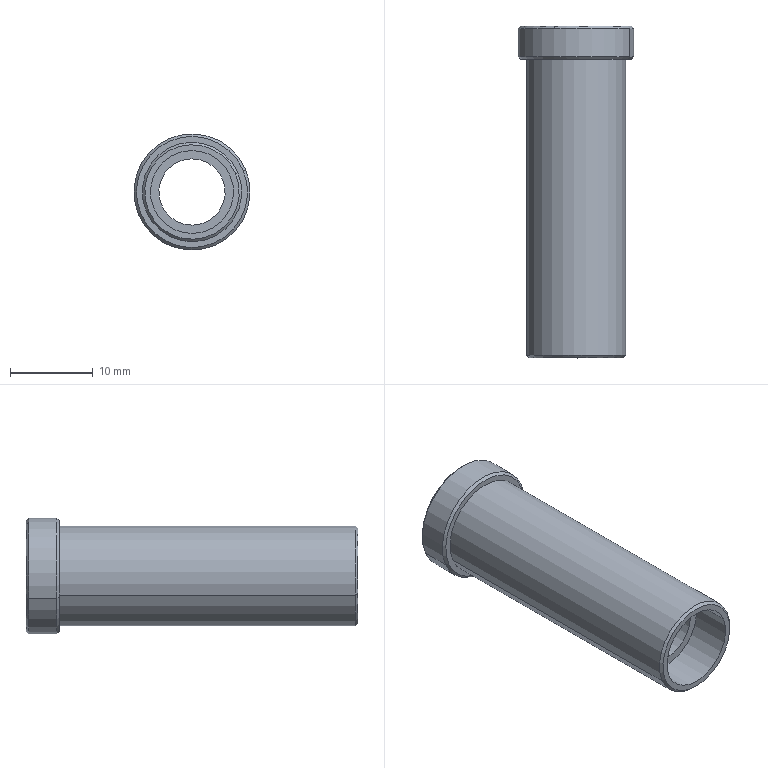Component | SolidWorks | 04LowerMaterialReceivingSwingAngleAssembly(3920)-1_EwellixBallBushingLOC71-D8-L40-E40-G30-7_LOC71-D8-L40-E40-G30-2-1 | 1 solid | 21 faces | box 14 x 40 x 14 mm | volume 2388 mm3 | cylinder 10 | cone 6 | plane 5 | commonest cylinder face diameters 10 x4 12 x2 14 x2 8 x2
STEP:
#1=CARTESIAN_POINT('',(-4.662,5.201,11.122));
#2=VERTEX_POINT('',#1);
#3=CARTESIAN_POINT('',(-5.099,5.201,10.941));
#4=VERTEX_POINT('',#3);
#5=CARTESIAN_POINT('',(-4.88,5.201,11.031));
#6=DIRECTION('',(0.,1.,0.));
#7=DIRECTION('',(0.9237,0.,0.3832));
#8=AXIS2_PLACEMENT_3D('',#5,#6,#7);
#9=CIRCLE('',#8,0.2362);
#10=EDGE_CURVE('',#2,#4,#9,.T.);
#11=ORIENTED_EDGE('',*,*,#10,.T.);
#12=CARTESIAN_POINT('',(-5.099,6.607,10.941));
#13=VERTEX_POINT('',#12);
#14=CARTESIAN_POINT('',(-5.099,-12.921,10.941));
#15=DIRECTION('',(0.,1.,0.));
#16=VECTOR('',#15,39.37);
#17=LINE('',#14,#16);
#18=EDGE_CURVE('',#4,#13,#17,.T.);
#19=ORIENTED_EDGE('',*,*,#18,.T.);
#20=CARTESIAN_POINT('',(-4.662,6.607,11.122));
#21=VERTEX_POINT('',#20);
#22=CARTESIAN_POINT('',(-4.88,6.607,11.031));
#23=DIRECTION('',(-0.,-1.,-0.));
#24=DIRECTION('',(0.9237,0.,0.3832));
#25=AXIS2_PLACEMENT_3D('',#22,#23,#24);
#26=CIRCLE('',#25,0.2362);
#27=EDGE_CURVE('',#13,#21,#26,.T.);
#28=ORIENTED_EDGE('',*,*,#27,.T.);
#29=CARTESIAN_POINT('',(-4.662,-12.921,11.122));
#30=DIRECTION('',(0.,1.,0.));
#31=VECTOR('',#30,39.37);
#32=LINE('',#29,#31);
#33=EDGE_CURVE('',#2,#21,#32,.T.);
#34=ORIENTED_EDGE('',*,*,#33,.F.);
#35=EDGE_LOOP('',(#11,#19,#28,#34));
#36=FACE_OUTER_BOUND('',#35,.T.);
#37=CARTESIAN_POINT('',(-4.88,-12.921,11.031));
#38=DIRECTION('',(0.,1.,0.));
#39=DIRECTION('',(0.9237,0.,0.3832));
#40=AXIS2_PLACEMENT_3D('',#37,#38,#39);
#41=CYLINDRICAL_SURFACE('',#40,0.2362);
#42=ADVANCED_FACE('',(#36),#41,.T.);
#43=CARTESIAN_POINT('',(-4.673,5.189,11.117));
#44=VERTEX_POINT('',#43);
#45=CARTESIAN_POINT('',(-5.088,5.189,10.945));
#46=VERTEX_POINT('',#45);
#47=CARTESIAN_POINT('',(-4.88,5.189,11.031));
#48=DIRECTION('',(0.,1.,0.));
#49=DIRECTION('',(0.9237,0.,0.3832));
#50=AXIS2_PLACEMENT_3D('',#47,#48,#49);
#51=CIRCLE('',#50,0.2244);
#52=EDGE_CURVE('',#44,#46,#51,.T.);
#53=ORIENTED_EDGE('',*,*,#52,.T.);
#54=CARTESIAN_POINT('',(-5.099,5.201,10.941));
#55=DIRECTION('',(-0.6531,0.7071,-0.271));
#56=VECTOR('',#55,39.37);
#57=LINE('',#54,#56);
#58=EDGE_CURVE('',#46,#4,#57,.T.);
#59=ORIENTED_EDGE('',*,*,#58,.T.);
#60=ORIENTED_EDGE('',*,*,#10,.F.);
#61=CARTESIAN_POINT('',(-4.662,5.201,11.122));
#62=DIRECTION('',(0.6531,0.7071,0.271));
#63=VECTOR('',#62,39.37);
#64=LINE('',#61,#63);
#65=EDGE_CURVE('',#44,#2,#64,.T.);
#66=ORIENTED_EDGE('',*,*,#65,.F.);
#67=EDGE_LOOP('',(#53,#59,#60,#66));
#68=FACE_OUTER_BOUND('',#67,.T.);
#69=CARTESIAN_POINT('',(-4.88,5.201,11.031));
#70=DIRECTION('',(0.,1.,0.));
#71=DIRECTION('',(0.9237,0.,0.3832));
#72=AXIS2_PLACEMENT_3D('',#69,#70,#71);
#73=CONICAL_SURFACE('',#72,0.2362,0.7854);
#74=ADVANCED_FACE('',(#68),#73,.T.);
#75=CARTESIAN_POINT('',(-5.124,6.607,10.93));
#76=VERTEX_POINT('',#75);
#77=CARTESIAN_POINT('',(-4.637,6.607,11.132));
#78=VERTEX_POINT('',#77);
#79=CARTESIAN_POINT('',(-4.88,6.607,11.031));
#80=DIRECTION('',(-0.,-1.,-0.));
#81=DIRECTION('',(0.9237,0.,0.3832));
#82=AXIS2_PLACEMENT_3D('',#79,#80,#81);
#83=CIRCLE('',#82,0.2638);
#84=EDGE_CURVE('',#76,#78,#83,.T.);
#85=ORIENTED_EDGE('',*,*,#84,.F.);
#86=CARTESIAN_POINT('',(-5.135,6.619,10.926));
#87=VERTEX_POINT('',#86);
#88=CARTESIAN_POINT('',(-5.135,6.619,10.926));
#89=DIRECTION('',(-0.6531,0.7071,-0.271));
#90=VECTOR('',#89,39.37);
#91=LINE('',#88,#90);
#92=EDGE_CURVE('',#76,#87,#91,.T.);
#93=ORIENTED_EDGE('',*,*,#92,.T.);
#94=CARTESIAN_POINT('',(-4.626,6.619,11.137));
#95=VERTEX_POINT('',#94);
#96=CARTESIAN_POINT('',(-4.88,6.619,11.031));
#97=DIRECTION('',(-0.,-1.,-0.));
#98=DIRECTION('',(0.9237,0.,0.3832));
#99=AXIS2_PLACEMENT_3D('',#96,#97,#98);
#100=CIRCLE('',#99,0.2756);
#101=EDGE_CURVE('',#87,#95,#100,.T.);
#102=ORIENTED_EDGE('',*,*,#101,.T.);
#103=CARTESIAN_POINT('',(-4.626,6.619,11.137));
#104=DIRECTION('',(0.6531,0.7071,0.271));
#105=VECTOR('',#104,39.37);
#106=LINE('',#103,#105);
#107=EDGE_CURVE('',#78,#95,#106,.T.);
#108=ORIENTED_EDGE('',*,*,#107,.F.);
#109=EDGE_LOOP('',(#85,#93,#102,#108));
#110=FACE_OUTER_BOUND('',#109,.T.);
#111=CARTESIAN_POINT('',(-4.88,6.619,11.031));
#112=DIRECTION('',(0.,1.,0.));
#113=DIRECTION('',(0.9237,0.,0.3832));
#114=AXIS2_PLACEMENT_3D('',#111,#112,#113);
#115=CONICAL_SURFACE('',#114,0.2756,0.7854);
#116=ADVANCED_FACE('',(#110),#115,.T.);
#117=CARTESIAN_POINT('',(-5.062,5.189,10.956));
#118=VERTEX_POINT('',#117);
#119=CARTESIAN_POINT('',(-4.699,5.189,11.107));
#120=VERTEX_POINT('',#119);
#121=CARTESIAN_POINT('',(-4.88,5.189,11.031));
#122=DIRECTION('',(0.,1.,0.));
#123=DIRECTION('',(0.9237,0.,0.3832));
#124=AXIS2_PLACEMENT_3D('',#121,#122,#123);
#125=CIRCLE('',#124,0.1969);
#126=EDGE_CURVE('',#118,#120,#125,.T.);
#127=ORIENTED_EDGE('',*,*,#126,.F.);
#128=CARTESIAN_POINT('',(-5.062,5.386,10.956));
#129=VERTEX_POINT('',#128);
#130=CARTESIAN_POINT('',(-5.062,-12.921,10.956));
#131=DIRECTION('',(0.,1.,0.));
#132=VECTOR('',#131,39.37);
#133=LINE('',#130,#132);
#134=EDGE_CURVE('',#118,#129,#133,.T.);
#135=ORIENTED_EDGE('',*,*,#134,.T.);
#136=CARTESIAN_POINT('',(-4.699,5.386,11.107));
#137=VERTEX_POINT('',#136);
#138=CARTESIAN_POINT('',(-4.88,5.386,11.031));
#139=DIRECTION('',(-0.,-1.,-0.));
#140=DIRECTION('',(0.9237,0.,0.3832));
#141=AXIS2_PLACEMENT_3D('',#138,#139,#140);
#142=CIRCLE('',#141,0.1969);
#143=EDGE_CURVE('',#137,#129,#142,.T.);
#144=ORIENTED_EDGE('',*,*,#143,.F.);
#145=CARTESIAN_POINT('',(-4.699,-12.921,11.107));
#146=DIRECTION('',(0.,1.,0.));
#147=VECTOR('',#146,39.37);
#148=LINE('',#145,#147);
#149=EDGE_CURVE('',#120,#137,#148,.T.);
#150=ORIENTED_EDGE('',*,*,#149,.F.);
#151=EDGE_LOOP('',(#127,#135,#144,#150));
#152=FACE_OUTER_BOUND('',#151,.T.);
#153=CARTESIAN_POINT('',(-4.88,-12.921,11.031));
#154=DIRECTION('',(0.,1.,0.));
#155=DIRECTION('',(0.9237,0.,0.3832));
#156=AXIS2_PLACEMENT_3D('',#153,#154,#155);
#157=CYLINDRICAL_SURFACE('',#156,0.1969);
#158=ADVANCED_FACE('',(#152),#157,.F.);
#159=ORIENTED_EDGE('',*,*,#101,.F.);
#160=CARTESIAN_POINT('',(-5.135,6.752,10.926));
#161=VERTEX_POINT('',#160);
#162=CARTESIAN_POINT('',(-5.135,-12.921,10.926));
#163=DIRECTION('',(0.,1.,0.));
#164=VECTOR('',#163,39.37);
#165=LINE('',#162,#164);
#166=EDGE_CURVE('',#87,#161,#165,.T.);
#167=ORIENTED_EDGE('',*,*,#166,.T.);
#168=CARTESIAN_POINT('',(-4.775,6.752,10.777));
#169=VERTEX_POINT('',#168);
#170=CARTESIAN_POINT('',(-4.88,6.752,11.031));
#171=DIRECTION('',(-0.,-1.,-0.));
#172=DIRECTION('',(0.9237,0.,0.3832));
#173=AXIS2_PLACEMENT_3D('',#170,#171,#172);
#174=CIRCLE('',#173,0.2756);
#175=EDGE_CURVE('',#161,#169,#174,.T.);
#176=ORIENTED_EDGE('',*,*,#175,.T.);
#177=CARTESIAN_POINT('',(-4.626,6.752,11.137));
#178=VERTEX_POINT('',#177);
#179=CARTESIAN_POINT('',(-4.88,6.752,11.031));
#180=DIRECTION('',(-0.,-1.,-0.));
#181=DIRECTION('',(0.9237,0.,0.3832));
#182=AXIS2_PLACEMENT_3D('',#179,#180,#181);
#183=CIRCLE('',#182,0.2756);
#184=EDGE_CURVE('',#169,#178,#183,.T.);
#185=ORIENTED_EDGE('',*,*,#184,.T.);
#186=CARTESIAN_POINT('',(-4.626,-12.921,11.137));
#187=DIRECTION('',(0.,1.,0.));
#188=VECTOR('',#187,39.37);
#189=LINE('',#186,#188);
#190=EDGE_CURVE('',#95,#178,#189,.T.);
#191=ORIENTED_EDGE('',*,*,#190,.F.);
#192=EDGE_LOOP('',(#159,#167,#176,#185,#191));
#193=FACE_OUTER_BOUND('',#192,.T.);
#194=CARTESIAN_POINT('',(-4.88,-12.921,11.031));
#195=DIRECTION('',(0.,1.,0.));
#196=DIRECTION('',(0.9237,0.,0.3832));
#197=AXIS2_PLACEMENT_3D('',#194,#195,#196);
#198=CYLINDRICAL_SURFACE('',#197,0.2756);
#199=ADVANCED_FACE('',(#193),#198,.T.);
#200=CARTESIAN_POINT('',(-4.779,6.764,10.788));
#201=VERTEX_POINT('',#200);
#202=CARTESIAN_POINT('',(-4.982,6.764,11.275));
#203=VERTEX_POINT('',#202);
#204=CARTESIAN_POINT('',(-4.88,6.764,11.031));
#205=DIRECTION('',(0.,-1.,-0.));
#206=DIRECTION('',(0.3832,0.,-0.9237));
#207=AXIS2_PLACEMENT_3D('',#204,#205,#206);
#208=CIRCLE('',#207,0.2638);
#209=EDGE_CURVE('',#201,#203,#208,.T.);
#210=ORIENTED_EDGE('',*,*,#209,.T.);
#211=CARTESIAN_POINT('',(-4.986,6.752,11.286));
#212=VERTEX_POINT('',#211);
#213=CARTESIAN_POINT('',(-4.986,6.752,11.286));
#214=DIRECTION('',(-0.271,-0.7071,0.6531));
#215=VECTOR('',#214,39.37);
#216=LINE('',#213,#215);
#217=EDGE_CURVE('',#203,#212,#216,.T.);
#218=ORIENTED_EDGE('',*,*,#217,.T.);
#219=CARTESIAN_POINT('',(-4.88,6.752,11.031));
#220=DIRECTION('',(-0.,-1.,-0.));
#221=DIRECTION('',(0.9237,0.,0.3832));
#222=AXIS2_PLACEMENT_3D('',#219,#220,#221);
#223=CIRCLE('',#222,0.2756);
#224=EDGE_CURVE('',#178,#212,#223,.T.);
#225=ORIENTED_EDGE('',*,*,#224,.F.);
#226=ORIENTED_EDGE('',*,*,#184,.F.);
#227=CARTESIAN_POINT('',(-4.775,6.752,10.777));
#228=DIRECTION('',(0.271,-0.7071,-0.6531));
#229=VECTOR('',#228,39.37);
#230=LINE('',#227,#229);
#231=EDGE_CURVE('',#201,#169,#230,.T.);
#232=ORIENTED_EDGE('',*,*,#231,.F.);
#233=EDGE_LOOP('',(#210,#218,#225,#226,#232));
#234=FACE_OUTER_BOUND('',#233,.T.);
#235=CARTESIAN_POINT('',(-4.88,6.752,11.031));
#236=DIRECTION('',(0.,-1.,-0.));
#237=DIRECTION('',(0.3832,0.,-0.9237));
#238=AXIS2_PLACEMENT_3D('',#235,#236,#237);
#239=CONICAL_SURFACE('',#238,0.2756,0.7854);
#240=ADVANCED_FACE('',(#234),#239,.T.);
#241=CARTESIAN_POINT('',(-5.026,5.386,10.971));
#242=VERTEX_POINT('',#241);
#243=CARTESIAN_POINT('',(-4.735,5.386,11.092));
#244=VERTEX_POINT('',#243);
#245=CARTESIAN_POINT('',(-4.88,5.386,11.031));
#246=DIRECTION('',(0.,1.,0.));
#247=DIRECTION('',(0.9237,0.,0.3832));
#248=AXIS2_PLACEMENT_3D('',#245,#246,#247);
#249=CIRCLE('',#248,0.1575);
#250=EDGE_CURVE('',#242,#244,#249,.T.);
#251=ORIENTED_EDGE('',*,*,#250,.F.);
#252=CARTESIAN_POINT('',(-5.026,6.567,10.971));
#253=VERTEX_POINT('',#252);
#254=CARTESIAN_POINT('',(-5.026,-12.921,10.971));
#255=DIRECTION('',(0.,1.,0.));
#256=VECTOR('',#255,39.37);
#257=LINE('',#254,#256);
#258=EDGE_CURVE('',#242,#253,#257,.T.);
#259=ORIENTED_EDGE('',*,*,#258,.T.);
#260=CARTESIAN_POINT('',(-4.735,6.567,11.092));
#261=VERTEX_POINT('',#260);
#262=CARTESIAN_POINT('',(-4.88,6.567,11.031));
#263=DIRECTION('',(-0.,-1.,-0.));
#264=DIRECTION('',(0.9237,0.,0.3832));
#265=AXIS2_PLACEMENT_3D('',#262,#263,#264);
#266=CIRCLE('',#265,0.1575);
#267=EDGE_CURVE('',#261,#253,#266,.T.);
#268=ORIENTED_EDGE('',*,*,#267,.F.);
#269=CARTESIAN_POINT('',(-4.735,-12.921,11.092));
#270=DIRECTION('',(0.,1.,0.));
#271=VECTOR('',#270,39.37);
#272=LINE('',#269,#271);
#273=EDGE_CURVE('',#244,#261,#272,.T.);
#274=ORIENTED_EDGE('',*,*,#273,.F.);
#275=EDGE_LOOP('',(#251,#259,#268,#274));
#276=FACE_OUTER_BOUND('',#275,.T.);
#277=CARTESIAN_POINT('',(-4.88,-12.921,11.031));
#278=DIRECTION('',(0.,1.,0.));
#279=DIRECTION('',(0.9237,0.,0.3832));
#280=AXIS2_PLACEMENT_3D('',#277,#278,#279);
#281=CYLINDRICAL_SURFACE('',#280,0.1575);
#282=ADVANCED_FACE('',(#276),#281,.F.);
#283=CARTESIAN_POINT('',(-5.062,6.567,10.956));
#284=VERTEX_POINT('',#283);
#285=CARTESIAN_POINT('',(-4.699,6.567,11.107));
#286=VERTEX_POINT('',#285);
#287=CARTESIAN_POINT('',(-4.88,6.567,11.031));
#288=DIRECTION('',(0.,1.,0.));
#289=DIRECTION('',(0.9237,0.,0.3832));
#290=AXIS2_PLACEMENT_3D('',#287,#288,#289);
#291=CIRCLE('',#290,0.1969);
#292=EDGE_CURVE('',#284,#286,#291,.T.);
#293=ORIENTED_EDGE('',*,*,#292,.F.);
#294=CARTESIAN_POINT('',(-5.062,6.764,10.956));
#295=VERTEX_POINT('',#294);
#296=CARTESIAN_POINT('',(-5.062,-12.921,10.956));
#297=DIRECTION('',(0.,1.,0.));
#298=VECTOR('',#297,39.37);
#299=LINE('',#296,#298);
#300=EDGE_CURVE('',#284,#295,#299,.T.);
#301=ORIENTED_EDGE('',*,*,#300,.T.);
#302=CARTESIAN_POINT('',(-4.699,6.764,11.107));
#303=VERTEX_POINT('',#302);
#304=CARTESIAN_POINT('',(-4.88,6.764,11.031));
#305=DIRECTION('',(-0.,-1.,-0.));
#306=DIRECTION('',(0.9237,0.,0.3832));
#307=AXIS2_PLACEMENT_3D('',#304,#305,#306);
#308=CIRCLE('',#307,0.1969);
#309=EDGE_CURVE('',#303,#295,#308,.T.);
#310=ORIENTED_EDGE('',*,*,#309,.F.);
#311=CARTESIAN_POINT('',(-4.699,-12.921,11.107));
#312=DIRECTION('',(0.,1.,0.));
#313=VECTOR('',#312,39.37);
#314=LINE('',#311,#313);
#315=EDGE_CURVE('',#286,#303,#314,.T.);
#316=ORIENTED_EDGE('',*,*,#315,.F.);
#317=EDGE_LOOP('',(#293,#301,#310,#316));
#318=FACE_OUTER_BOUND('',#317,.T.);
#319=CARTESIAN_POINT('',(-4.88,-12.921,11.031));
#320=DIRECTION('',(0.,1.,0.));
#321=DIRECTION('',(0.9237,0.,0.3832));
#322=AXIS2_PLACEMENT_3D('',#319,#320,#321);
#323=CYLINDRICAL_SURFACE('',#322,0.1969);
#324=ADVANCED_FACE('',(#318),#323,.F.);
#325=ORIENTED_EDGE('',*,*,#18,.F.);
#326=CARTESIAN_POINT('',(-4.88,5.201,11.031));
#327=DIRECTION('',(0.,1.,0.));
#328=DIRECTION('',(0.9237,0.,0.3832));
#329=AXIS2_PLACEMENT_3D('',#326,#327,#328);
#330=CIRCLE('',#329,0.2362);
#331=EDGE_CURVE('',#4,#2,#330,.T.);
#332=ORIENTED_EDGE('',*,*,#331,.T.);
#333=ORIENTED_EDGE('',*,*,#33,.T.);
#334=CARTESIAN_POINT('',(-4.88,6.607,11.031));
#335=DIRECTION('',(-0.,-1.,-0.));
#336=DIRECTION('',(0.9237,0.,0.3832));
#337=AXIS2_PLACEMENT_3D('',#334,#335,#336);
#338=CIRCLE('',#337,0.2362);
#339=EDGE_CURVE('',#21,#13,#338,.T.);
#340=ORIENTED_EDGE('',*,*,#339,.T.);
#341=EDGE_LOOP('',(#325,#332,#333,#340));
#342=FACE_OUTER_BOUND('',#341,.T.);
#343=CARTESIAN_POINT('',(-4.88,-12.921,11.031));
#344=DIRECTION('',(0.,1.,0.));
#345=DIRECTION('',(0.9237,0.,0.3832));
#346=AXIS2_PLACEMENT_3D('',#343,#344,#345);
#347=CYLINDRICAL_SURFACE('',#346,0.2362);
#348=ADVANCED_FACE('',(#342),#347,.T.);
#349=ORIENTED_EDGE('',*,*,#58,.F.);
#350=CARTESIAN_POINT('',(-4.88,5.189,11.031));
#351=DIRECTION('',(0.,1.,0.));
#352=DIRECTION('',(0.9237,0.,0.3832));
#353=AXIS2_PLACEMENT_3D('',#350,#351,#352);
#354=CIRCLE('',#353,0.2244);
#355=EDGE_CURVE('',#46,#44,#354,.T.);
#356=ORIENTED_EDGE('',*,*,#355,.T.);
#357=ORIENTED_EDGE('',*,*,#65,.T.);
#358=ORIENTED_EDGE('',*,*,#331,.F.);
#359=EDGE_LOOP('',(#349,#356,#357,#358));
#360=FACE_OUTER_BOUND('',#359,.T.);
#361=CARTESIAN_POINT('',(-4.88,5.201,11.031));
#362=DIRECTION('',(0.,1.,0.));
#363=DIRECTION('',(0.9237,0.,0.3832));
#364=AXIS2_PLACEMENT_3D('',#361,#362,#363);
#365=CONICAL_SURFACE('',#364,0.2362,0.7854);
#366=ADVANCED_FACE('',(#360),#365,.T.);
#367=ORIENTED_EDGE('',*,*,#339,.F.);
#368=ORIENTED_EDGE('',*,*,#27,.F.);
#369=EDGE_LOOP('',(#367,#368));
#370=FACE_BOUND('',#369,.T.);
#371=CARTESIAN_POINT('',(-4.88,6.607,11.031));
#372=DIRECTION('',(-0.,-1.,-0.));
#373=DIRECTION('',(0.9237,0.,0.3832));
#374=AXIS2_PLACEMENT_3D('',#371,#372,#373);
#375=CIRCLE('',#374,0.2638);
#376=EDGE_CURVE('',#78,#76,#375,.T.);
#377=ORIENTED_EDGE('',*,*,#376,.T.);
#378=ORIENTED_EDGE('',*,*,#84,.T.);
#379=EDGE_LOOP('',(#377,#378));
#380=FACE_OUTER_BOUND('',#379,.T.);
#381=CARTESIAN_POINT('',(-4.79,6.607,10.813));
#382=DIRECTION('',(-0.,-1.,-0.));
#383=DIRECTION('',(-0.9237,0.,-0.3832));
#384=AXIS2_PLACEMENT_3D('',#381,#382,#383);
#385=PLANE('',#384);
#386=ADVANCED_FACE('',(#370,#380),#385,.T.);
#387=CARTESIAN_POINT('',(-4.88,5.189,11.031));
#388=DIRECTION('',(0.,1.,0.));
#389=DIRECTION('',(0.9237,0.,0.3832));
#390=AXIS2_PLACEMENT_3D('',#387,#388,#389);
#391=CIRCLE('',#390,0.1969);
#392=EDGE_CURVE('',#120,#118,#391,.T.);
#393=ORIENTED_EDGE('',*,*,#392,.T.);
#394=ORIENTED_EDGE('',*,*,#126,.T.);
#395=EDGE_LOOP('',(#393,#394));
#396=FACE_BOUND('',#395,.T.);
#397=ORIENTED_EDGE('',*,*,#52,.F.);
#398=ORIENTED_EDGE('',*,*,#355,.F.);
#399=EDGE_LOOP('',(#397,#398));
#400=FACE_OUTER_BOUND('',#399,.T.);
#401=CARTESIAN_POINT('',(-4.805,5.189,10.85));
#402=DIRECTION('',(-0.,-1.,-0.));
#403=DIRECTION('',(-0.9237,0.,-0.3832));
#404=AXIS2_PLACEMENT_3D('',#401,#402,#403);
#405=PLANE('',#404);
#406=ADVANCED_FACE('',(#396,#400),#405,.T.);
#407=ORIENTED_EDGE('',*,*,#92,.F.);
#408=ORIENTED_EDGE('',*,*,#376,.F.);
#409=ORIENTED_EDGE('',*,*,#107,.T.);
#410=CARTESIAN_POINT('',(-4.88,6.619,11.031));
#411=DIRECTION('',(-0.,-1.,-0.));
#412=DIRECTION('',(0.9237,0.,0.3832));
#413=AXIS2_PLACEMENT_3D('',#410,#411,#412);
#414=CIRCLE('',#413,0.2756);
#415=EDGE_CURVE('',#95,#87,#414,.T.);
#416=ORIENTED_EDGE('',*,*,#415,.T.);
#417=EDGE_LOOP('',(#407,#408,#409,#416));
#418=FACE_OUTER_BOUND('',#417,.T.);
#419=CARTESIAN_POINT('',(-4.88,6.619,11.031));
#420=DIRECTION('',(0.,1.,0.));
#421=DIRECTION('',(0.9237,0.,0.3832));
#422=AXIS2_PLACEMENT_3D('',#419,#420,#421);
#423=CONICAL_SURFACE('',#422,0.2756,0.7854);
#424=ADVANCED_FACE('',(#418),#423,.T.);
#425=ORIENTED_EDGE('',*,*,#134,.F.);
#426=ORIENTED_EDGE('',*,*,#392,.F.);
#427=ORIENTED_EDGE('',*,*,#149,.T.);
#428=CARTESIAN_POINT('',(-4.88,5.386,11.031));
#429=DIRECTION('',(-0.,-1.,-0.));
#430=DIRECTION('',(0.9237,0.,0.3832));
#431=AXIS2_PLACEMENT_3D('',#428,#429,#430);
#432=CIRCLE('',#431,0.1969);
#433=EDGE_CURVE('',#129,#137,#432,.T.);
#434=ORIENTED_EDGE('',*,*,#433,.F.);
#435=EDGE_LOOP('',(#425,#426,#427,#434));
#436=FACE_OUTER_BOUND('',#435,.T.);
#437=CARTESIAN_POINT('',(-4.88,-12.921,11.031));
#438=DIRECTION('',(0.,1.,0.));
#439=DIRECTION('',(0.9237,0.,0.3832));
#440=AXIS2_PLACEMENT_3D('',#437,#438,#439);
#441=CYLINDRICAL_SURFACE('',#440,0.1969);
#442=ADVANCED_FACE('',(#436),#441,.F.);
#443=ORIENTED_EDGE('',*,*,#166,.F.);
#444=ORIENTED_EDGE('',*,*,#415,.F.);
#445=ORIENTED_EDGE('',*,*,#190,.T.);
#446=ORIENTED_EDGE('',*,*,#224,.T.);
#447=CARTESIAN_POINT('',(-4.88,6.752,11.031));
#448=DIRECTION('',(-0.,-1.,-0.));
#449=DIRECTION('',(0.9237,0.,0.3832));
#450=AXIS2_PLACEMENT_3D('',#447,#448,#449);
#451=CIRCLE('',#450,0.2756);
#452=EDGE_CURVE('',#212,#161,#451,.T.);
#453=ORIENTED_EDGE('',*,*,#452,.T.);
#454=EDGE_LOOP('',(#443,#444,#445,#446,#453));
#455=FACE_OUTER_BOUND('',#454,.T.);
#456=CARTESIAN_POINT('',(-4.88,-12.921,11.031));
#457=DIRECTION('',(0.,1.,0.));
#458=DIRECTION('',(0.9237,0.,0.3832));
#459=AXIS2_PLACEMENT_3D('',#456,#457,#458);
#460=CYLINDRICAL_SURFACE('',#459,0.2756);
#461=ADVANCED_FACE('',(#455),#460,.T.);
#462=CARTESIAN_POINT('',(-4.88,5.386,11.031));
#463=DIRECTION('',(0.,1.,0.));
#464=DIRECTION('',(0.9237,0.,0.3832));
#465=AXIS2_PLACEMENT_3D('',#462,#463,#464);
#466=CIRCLE('',#465,0.1575);
#467=EDGE_CURVE('',#244,#242,#466,.T.);
#468=ORIENTED_EDGE('',*,*,#467,.T.);
#469=ORIENTED_EDGE('',*,*,#250,.T.);
#470=EDGE_LOOP('',(#468,#469));
#471=FACE_BOUND('',#470,.T.);
#472=ORIENTED_EDGE('',*,*,#143,.T.);
#473=ORIENTED_EDGE('',*,*,#433,.T.);
#474=EDGE_LOOP('',(#472,#473));
#475=FACE_OUTER_BOUND('',#474,.T.);
#476=CARTESIAN_POINT('',(-4.82,5.386,10.886));
#477=DIRECTION('',(-0.,-1.,-0.));
#478=DIRECTION('',(-0.9237,0.,-0.3832));
#479=AXIS2_PLACEMENT_3D('',#476,#477,#478);
#480=PLANE('',#479);
#481=ADVANCED_FACE('',(#471,#475),#480,.T.);
#482=ORIENTED_EDGE('',*,*,#217,.F.);
#483=CARTESIAN_POINT('',(-4.88,6.764,11.031));
#484=DIRECTION('',(0.,-1.,-0.));
#485=DIRECTION('',(0.3832,0.,-0.9237));
#486=AXIS2_PLACEMENT_3D('',#483,#484,#485);
#487=CIRCLE('',#486,0.2638);
#488=EDGE_CURVE('',#203,#201,#487,.T.);
#489=ORIENTED_EDGE('',*,*,#488,.T.);
#490=ORIENTED_EDGE('',*,*,#231,.T.);
#491=ORIENTED_EDGE('',*,*,#175,.F.);
#492=ORIENTED_EDGE('',*,*,#452,.F.);
#493=EDGE_LOOP('',(#482,#489,#490,#491,#492));
#494=FACE_OUTER_BOUND('',#493,.T.);
#495=CARTESIAN_POINT('',(-4.88,6.752,11.031));
#496=DIRECTION('',(0.,-1.,-0.));
#497=DIRECTION('',(0.3832,0.,-0.9237));
#498=AXIS2_PLACEMENT_3D('',#495,#496,#497);
#499=CONICAL_SURFACE('',#498,0.2756,0.7854);
#500=ADVANCED_FACE('',(#494),#499,.T.);
#501=ORIENTED_EDGE('',*,*,#258,.F.);
#502=ORIENTED_EDGE('',*,*,#467,.F.);
#503=ORIENTED_EDGE('',*,*,#273,.T.);
#504=CARTESIAN_POINT('',(-4.88,6.567,11.031));
#505=DIRECTION('',(-0.,-1.,-0.));
#506=DIRECTION('',(0.9237,0.,0.3832));
#507=AXIS2_PLACEMENT_3D('',#504,#505,#506);
#508=CIRCLE('',#507,0.1575);
#509=EDGE_CURVE('',#253,#261,#508,.T.);
#510=ORIENTED_EDGE('',*,*,#509,.F.);
#511=EDGE_LOOP('',(#501,#502,#503,#510));
#512=FACE_OUTER_BOUND('',#511,.T.);
#513=CARTESIAN_POINT('',(-4.88,-12.921,11.031));
#514=DIRECTION('',(0.,1.,0.));
#515=DIRECTION('',(0.9237,0.,0.3832));
#516=AXIS2_PLACEMENT_3D('',#513,#514,#515);
#517=CYLINDRICAL_SURFACE('',#516,0.1575);
#518=ADVANCED_FACE('',(#512),#517,.F.);
#519=ORIENTED_EDGE('',*,*,#209,.F.);
#520=ORIENTED_EDGE('',*,*,#488,.F.);
#521=EDGE_LOOP('',(#519,#520));
#522=FACE_OUTER_BOUND('',#521,.T.);
#523=ORIENTED_EDGE('',*,*,#309,.T.);
#524=CARTESIAN_POINT('',(-4.88,6.764,11.031));
#525=DIRECTION('',(-0.,-1.,-0.));
#526=DIRECTION('',(0.9237,0.,0.3832));
#527=AXIS2_PLACEMENT_3D('',#524,#525,#526);
#528=CIRCLE('',#527,0.1969);
#529=EDGE_CURVE('',#295,#303,#528,.T.);
#530=ORIENTED_EDGE('',*,*,#529,.T.);
#531=EDGE_LOOP('',(#523,#530));
#532=FACE_BOUND('',#531,.T.);
#533=CARTESIAN_POINT('',(-4.779,6.764,10.788));
#534=DIRECTION('',(0.,1.,0.));
#535=DIRECTION('',(0.9237,-0.,0.3832));
#536=AXIS2_PLACEMENT_3D('',#533,#534,#535);
#537=PLANE('',#536);
#538=ADVANCED_FACE('',(#522,#532),#537,.T.);
#539=CARTESIAN_POINT('',(-4.88,6.567,11.031));
#540=DIRECTION('',(0.,1.,0.));
#541=DIRECTION('',(0.9237,0.,0.3832));
#542=AXIS2_PLACEMENT_3D('',#539,#540,#541);
#543=CIRCLE('',#542,0.1969);
#544=EDGE_CURVE('',#286,#284,#543,.T.);
#545=ORIENTED_EDGE('',*,*,#544,.T.);
#546=ORIENTED_EDGE('',*,*,#292,.T.);
#547=EDGE_LOOP('',(#545,#546));
#548=FACE_OUTER_BOUND('',#547,.T.);
#549=ORIENTED_EDGE('',*,*,#267,.T.);
#550=ORIENTED_EDGE('',*,*,#509,.T.);
#551=EDGE_LOOP('',(#549,#550));
#552=FACE_BOUND('',#551,.T.);
#553=CARTESIAN_POINT('',(-4.805,6.567,10.85));
#554=DIRECTION('',(0.,1.,0.));
#555=DIRECTION('',(0.9237,-0.,0.3832));
#556=AXIS2_PLACEMENT_3D('',#553,#554,#555);
#557=PLANE('',#556);
#558=ADVANCED_FACE('',(#548,#552),#557,.T.);
#559=ORIENTED_EDGE('',*,*,#300,.F.);
#560=ORIENTED_EDGE('',*,*,#544,.F.);
#561=ORIENTED_EDGE('',*,*,#315,.T.);
#562=ORIENTED_EDGE('',*,*,#529,.F.);
#563=EDGE_LOOP('',(#559,#560,#561,#562));
#564=FACE_OUTER_BOUND('',#563,.T.);
#565=CARTESIAN_POINT('',(-4.88,-12.921,11.031));
#566=DIRECTION('',(0.,1.,0.));
#567=DIRECTION('',(0.9237,0.,0.3832));
#568=AXIS2_PLACEMENT_3D('',#565,#566,#567);
#569=CYLINDRICAL_SURFACE('',#568,0.1969);
#570=ADVANCED_FACE('',(#564),#569,.F.);
#571=CLOSED_SHELL('',(#42,#74,#116,#158,#199,#240,#282,#324,#348,#366,#386,#406,#424,#442,#461,#481,#500,#518,#538,#558,#570));
#572=MANIFOLD_SOLID_BREP('',#571);
#573=CARTESIAN_POINT('',(0.,0.,0.));
#574=DIRECTION('',(0.,0.,1.));
#575=DIRECTION('',(1.,0.,0.));
#576=AXIS2_PLACEMENT_3D('',#573,#574,#575);
#577=(LENGTH_UNIT()NAMED_UNIT(*)SI_UNIT($,.METRE.));
#578=LENGTH_MEASURE_WITH_UNIT(LENGTH_MEASURE(0.0254),#577);
#579=DIMENSIONAL_EXPONENTS(1.,0.,0.,0.,0.,0.,0.);
#580=(CONVERSION_BASED_UNIT('',#578)LENGTH_UNIT()NAMED_UNIT(#579));
#581=UNCERTAINTY_MEASURE_WITH_UNIT(LENGTH_MEASURE(0.00001),#580,'','');
#582=(NAMED_UNIT(*)PLANE_ANGLE_UNIT()SI_UNIT($,.RADIAN.));
#583=(NAMED_UNIT(*)SI_UNIT($,.STERADIAN.)SOLID_ANGLE_UNIT());
#584=(GEOMETRIC_REPRESENTATION_CONTEXT(3)GLOBAL_UNCERTAINTY_ASSIGNED_CONTEXT((#581))GLOBAL_UNIT_ASSIGNED_CONTEXT((#580,#582,#583))REPRESENTATION_CONTEXT('',''));
#585=ADVANCED_BREP_SHAPE_REPRESENTATION('',(#572,#576),#584);
#586=COLOUR_RGB('',0.7922,0.8196,0.9333);
#587=FILL_AREA_STYLE_COLOUR('',#586);
#588=FILL_AREA_STYLE('',(#587));
#589=SURFACE_STYLE_FILL_AREA(#588);
#590=SURFACE_SIDE_STYLE('',(#589));
#591=SURFACE_STYLE_USAGE(.BOTH.,#590);
#592=PRESENTATION_STYLE_ASSIGNMENT((#591));
#593=STYLED_ITEM('',(#592),#572);
#594=PRESENTATION_LAYER_ASSIGNMENT('','',(#593));
#595=(LENGTH_UNIT()NAMED_UNIT(*)SI_UNIT($,.METRE.));
#596=LENGTH_MEASURE_WITH_UNIT(LENGTH_MEASURE(0.0254),#595);
#597=DIMENSIONAL_EXPONENTS(1.,0.,0.,0.,0.,0.,0.);
#598=(CONVERSION_BASED_UNIT('',#596)LENGTH_UNIT()NAMED_UNIT(#597));
#599=UNCERTAINTY_MEASURE_WITH_UNIT(LENGTH_MEASURE(0.00001),#598,'','');
#600=(NAMED_UNIT(*)PLANE_ANGLE_UNIT()SI_UNIT($,.RADIAN.));
#601=(NAMED_UNIT(*)SI_UNIT($,.STERADIAN.)SOLID_ANGLE_UNIT());
#602=(GEOMETRIC_REPRESENTATION_CONTEXT(3)GLOBAL_UNCERTAINTY_ASSIGNED_CONTEXT((#599))GLOBAL_UNIT_ASSIGNED_CONTEXT((#598,#600,#601))REPRESENTATION_CONTEXT('',''));
#603=MECHANICAL_DESIGN_GEOMETRIC_PRESENTATION_REPRESENTATION('',(#593),#602);